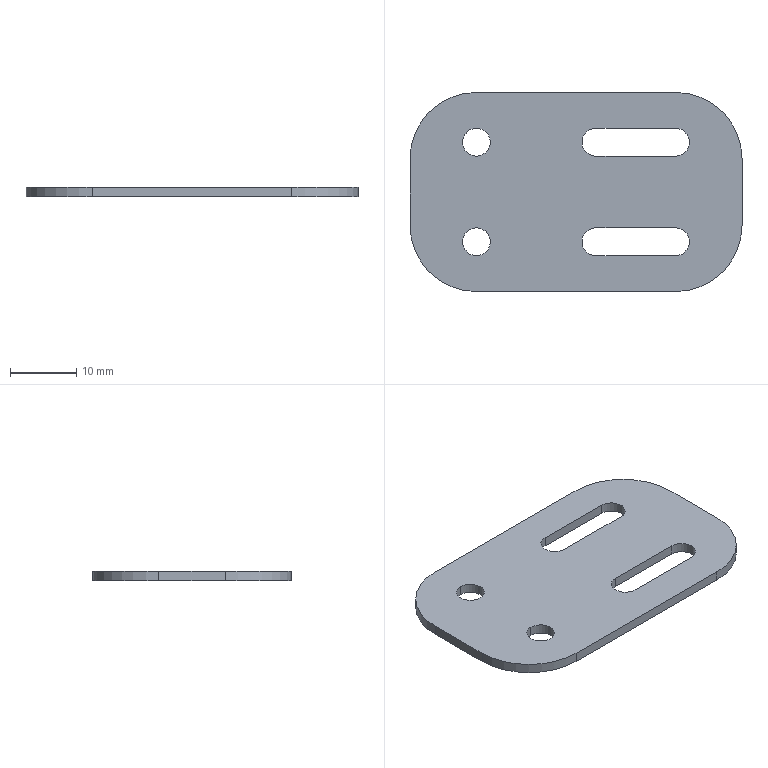CAM job | Mastercam | mm | 1 operations | part box 50 x 30 x 1.5
1. Contour (Ramp) | 3 - 3 平铣刀